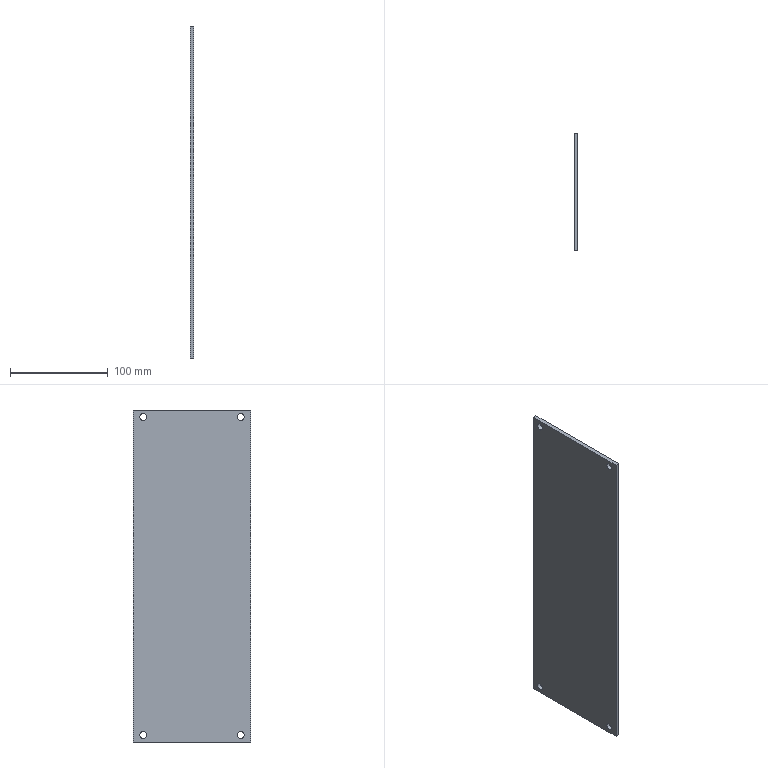Component | NX | HOUSING_COVER | 1 solid | 10 faces | box 4 x 120 x 340 mm | volume 162584 mm3 | plane 6 | cylinder 4 | commonest cylinder face diameters 7 x4
STEP:
#1=CARTESIAN_POINT('',(0.,0.,0.));
#2=DIRECTION('',(0.,0.,1.));
#3=DIRECTION('',(1.,0.,0.));
#4=AXIS2_PLACEMENT_3D('',#1,#2,#3);
#5=CARTESIAN_POINT('',(752.689,-210.302,-955.));
#6=VERTEX_POINT('',#5);
#7=CARTESIAN_POINT('',(752.689,-210.302,-1295.));
#8=VERTEX_POINT('',#7);
#9=CARTESIAN_POINT('',(752.689,-210.302,-955.));
#10=DIRECTION('',(0.,0.,-1.));
#11=VECTOR('',#10,1.);
#12=LINE('',#9,#11);
#13=CARTESIAN_POINT('',(756.689,-210.302,-955.));
#14=DIRECTION('',(0.,1.,0.));
#15=DIRECTION('',(-1.,0.,0.));
#16=AXIS2_PLACEMENT_3D('',#13,#14,#15);
#17=PLANE('',#16);
#18=CARTESIAN_POINT('',(4.,0.));
#19=DIRECTION('',(0.,-1.));
#20=VECTOR('',#19,1.);
#21=LINE('',#18,#20);
#22=(GEOMETRIC_REPRESENTATION_CONTEXT(2)PARAMETRIC_REPRESENTATION_CONTEXT()REPRESENTATION_CONTEXT('',''));
#23=DEFINITIONAL_REPRESENTATION('',(#21),#22);
#24=PCURVE('',#17,#23);
#25=CARTESIAN_POINT('',(752.689,-100.302,-962.));
#26=DIRECTION('',(-1.,0.,0.));
#27=DIRECTION('',(0.,-1.,0.));
#28=AXIS2_PLACEMENT_3D('',#25,#26,#27);
#29=PLANE('',#28);
#30=CARTESIAN_POINT('',(110.,7.));
#31=DIRECTION('',(0.,-1.));
#32=VECTOR('',#31,1.);
#33=LINE('',#30,#32);
#34=(GEOMETRIC_REPRESENTATION_CONTEXT(2)PARAMETRIC_REPRESENTATION_CONTEXT()REPRESENTATION_CONTEXT('',''));
#35=DEFINITIONAL_REPRESENTATION('',(#33),#34);
#36=PCURVE('',#29,#35);
#37=SURFACE_CURVE('',#12,(#24,#36),.PCURVE_S1.);
#38=EDGE_CURVE('',#6,#8,#37,.T.);
#39=ORIENTED_EDGE('',*,*,#38,.T.);
#40=CARTESIAN_POINT('',(756.689,-210.302,-1295.));
#41=VERTEX_POINT('',#40);
#42=CARTESIAN_POINT('',(756.689,-210.302,-1295.));
#43=DIRECTION('',(-1.,0.,0.));
#44=VECTOR('',#43,1.);
#45=LINE('',#42,#44);
#46=CARTESIAN_POINT('',(0.,-340.));
#47=DIRECTION('',(1.,0.));
#48=VECTOR('',#47,1.);
#49=LINE('',#46,#48);
#50=(GEOMETRIC_REPRESENTATION_CONTEXT(2)PARAMETRIC_REPRESENTATION_CONTEXT()REPRESENTATION_CONTEXT('',''));
#51=DEFINITIONAL_REPRESENTATION('',(#49),#50);
#52=PCURVE('',#17,#51);
#53=CARTESIAN_POINT('',(756.689,-210.302,-1295.));
#54=DIRECTION('',(0.,0.,1.));
#55=DIRECTION('',(1.,0.,0.));
#56=AXIS2_PLACEMENT_3D('',#53,#54,#55);
#57=PLANE('',#56);
#58=CARTESIAN_POINT('',(0.,0.));
#59=DIRECTION('',(-1.,0.));
#60=VECTOR('',#59,1.);
#61=LINE('',#58,#60);
#62=(GEOMETRIC_REPRESENTATION_CONTEXT(2)PARAMETRIC_REPRESENTATION_CONTEXT()REPRESENTATION_CONTEXT('',''));
#63=DEFINITIONAL_REPRESENTATION('',(#61),#62);
#64=PCURVE('',#57,#63);
#65=SURFACE_CURVE('',#45,(#52,#64),.PCURVE_S1.);
#66=EDGE_CURVE('',#41,#8,#65,.T.);
#67=ORIENTED_EDGE('',*,*,#66,.F.);
#68=CARTESIAN_POINT('',(756.689,-210.302,-955.));
#69=VERTEX_POINT('',#68);
#70=CARTESIAN_POINT('',(756.689,-210.302,-955.));
#71=DIRECTION('',(0.,0.,-1.));
#72=VECTOR('',#71,1.);
#73=LINE('',#70,#72);
#74=CARTESIAN_POINT('',(0.,0.));
#75=DIRECTION('',(0.,-1.));
#76=VECTOR('',#75,1.);
#77=LINE('',#74,#76);
#78=(GEOMETRIC_REPRESENTATION_CONTEXT(2)PARAMETRIC_REPRESENTATION_CONTEXT()REPRESENTATION_CONTEXT('',''));
#79=DEFINITIONAL_REPRESENTATION('',(#77),#78);
#80=PCURVE('',#17,#79);
#81=CARTESIAN_POINT('',(756.689,-100.302,-962.));
#82=DIRECTION('',(-1.,0.,0.));
#83=DIRECTION('',(0.,-1.,0.));
#84=AXIS2_PLACEMENT_3D('',#81,#82,#83);
#85=PLANE('',#84);
#86=CARTESIAN_POINT('',(110.,7.));
#87=DIRECTION('',(0.,-1.));
#88=VECTOR('',#87,1.);
#89=LINE('',#86,#88);
#90=(GEOMETRIC_REPRESENTATION_CONTEXT(2)PARAMETRIC_REPRESENTATION_CONTEXT()REPRESENTATION_CONTEXT('',''));
#91=DEFINITIONAL_REPRESENTATION('',(#89),#90);
#92=PCURVE('',#85,#91);
#93=SURFACE_CURVE('',#73,(#80,#92),.PCURVE_S1.);
#94=EDGE_CURVE('',#69,#41,#93,.T.);
#95=ORIENTED_EDGE('',*,*,#94,.F.);
#96=CARTESIAN_POINT('',(756.689,-210.302,-955.));
#97=DIRECTION('',(-1.,0.,0.));
#98=VECTOR('',#97,1.);
#99=LINE('',#96,#98);
#100=CARTESIAN_POINT('',(0.,0.));
#101=DIRECTION('',(1.,0.));
#102=VECTOR('',#101,1.);
#103=LINE('',#100,#102);
#104=(GEOMETRIC_REPRESENTATION_CONTEXT(2)PARAMETRIC_REPRESENTATION_CONTEXT()REPRESENTATION_CONTEXT('',''));
#105=DEFINITIONAL_REPRESENTATION('',(#103),#104);
#106=PCURVE('',#17,#105);
#107=CARTESIAN_POINT('',(756.689,-90.302,-955.));
#108=DIRECTION('',(0.,0.,-1.));
#109=DIRECTION('',(-1.,0.,0.));
#110=AXIS2_PLACEMENT_3D('',#107,#108,#109);
#111=PLANE('',#110);
#112=CARTESIAN_POINT('',(0.,-120.));
#113=DIRECTION('',(1.,0.));
#114=VECTOR('',#113,1.);
#115=LINE('',#112,#114);
#116=(GEOMETRIC_REPRESENTATION_CONTEXT(2)PARAMETRIC_REPRESENTATION_CONTEXT()REPRESENTATION_CONTEXT('',''));
#117=DEFINITIONAL_REPRESENTATION('',(#115),#116);
#118=PCURVE('',#111,#117);
#119=SURFACE_CURVE('',#99,(#106,#118),.PCURVE_S1.);
#120=EDGE_CURVE('',#69,#6,#119,.T.);
#121=ORIENTED_EDGE('',*,*,#120,.T.);
#122=EDGE_LOOP('',(#39,#67,#95,#121));
#123=FACE_BOUND('',#122,.T.);
#124=ADVANCED_FACE('',(#123),#17,.F.);
#125=CARTESIAN_POINT('',(752.689,-90.302,-1295.));
#126=VERTEX_POINT('',#125);
#127=CARTESIAN_POINT('',(752.689,-210.302,-1295.));
#128=DIRECTION('',(0.,1.,0.));
#129=VECTOR('',#128,1.);
#130=LINE('',#127,#129);
#131=CARTESIAN_POINT('',(-4.,0.));
#132=DIRECTION('',(0.,1.));
#133=VECTOR('',#132,1.);
#134=LINE('',#131,#133);
#135=(GEOMETRIC_REPRESENTATION_CONTEXT(2)PARAMETRIC_REPRESENTATION_CONTEXT()REPRESENTATION_CONTEXT('',''));
#136=DEFINITIONAL_REPRESENTATION('',(#134),#135);
#137=PCURVE('',#57,#136);
#138=CARTESIAN_POINT('',(110.,-333.));
#139=DIRECTION('',(-1.,0.));
#140=VECTOR('',#139,1.);
#141=LINE('',#138,#140);
#142=(GEOMETRIC_REPRESENTATION_CONTEXT(2)PARAMETRIC_REPRESENTATION_CONTEXT()REPRESENTATION_CONTEXT('',''));
#143=DEFINITIONAL_REPRESENTATION('',(#141),#142);
#144=PCURVE('',#29,#143);
#145=SURFACE_CURVE('',#130,(#137,#144),.PCURVE_S1.);
#146=EDGE_CURVE('',#8,#126,#145,.T.);
#147=ORIENTED_EDGE('',*,*,#146,.T.);
#148=CARTESIAN_POINT('',(756.689,-90.302,-1295.));
#149=VERTEX_POINT('',#148);
#150=CARTESIAN_POINT('',(756.689,-90.302,-1295.));
#151=DIRECTION('',(-1.,0.,0.));
#152=VECTOR('',#151,1.);
#153=LINE('',#150,#152);
#154=CARTESIAN_POINT('',(0.,120.));
#155=DIRECTION('',(-1.,0.));
#156=VECTOR('',#155,1.);
#157=LINE('',#154,#156);
#158=(GEOMETRIC_REPRESENTATION_CONTEXT(2)PARAMETRIC_REPRESENTATION_CONTEXT()REPRESENTATION_CONTEXT('',''));
#159=DEFINITIONAL_REPRESENTATION('',(#157),#158);
#160=PCURVE('',#57,#159);
#161=CARTESIAN_POINT('',(756.689,-90.302,-1295.));
#162=DIRECTION('',(0.,-1.,0.));
#163=DIRECTION('',(1.,0.,0.));
#164=AXIS2_PLACEMENT_3D('',#161,#162,#163);
#165=PLANE('',#164);
#166=CARTESIAN_POINT('',(0.,0.));
#167=DIRECTION('',(-1.,0.));
#168=VECTOR('',#167,1.);
#169=LINE('',#166,#168);
#170=(GEOMETRIC_REPRESENTATION_CONTEXT(2)PARAMETRIC_REPRESENTATION_CONTEXT()REPRESENTATION_CONTEXT('',''));
#171=DEFINITIONAL_REPRESENTATION('',(#169),#170);
#172=PCURVE('',#165,#171);
#173=SURFACE_CURVE('',#153,(#160,#172),.PCURVE_S1.);
#174=EDGE_CURVE('',#149,#126,#173,.T.);
#175=ORIENTED_EDGE('',*,*,#174,.F.);
#176=CARTESIAN_POINT('',(756.689,-210.302,-1295.));
#177=DIRECTION('',(0.,1.,0.));
#178=VECTOR('',#177,1.);
#179=LINE('',#176,#178);
#180=CARTESIAN_POINT('',(0.,0.));
#181=DIRECTION('',(0.,1.));
#182=VECTOR('',#181,1.);
#183=LINE('',#180,#182);
#184=(GEOMETRIC_REPRESENTATION_CONTEXT(2)PARAMETRIC_REPRESENTATION_CONTEXT()REPRESENTATION_CONTEXT('',''));
#185=DEFINITIONAL_REPRESENTATION('',(#183),#184);
#186=PCURVE('',#57,#185);
#187=CARTESIAN_POINT('',(110.,-333.));
#188=DIRECTION('',(-1.,0.));
#189=VECTOR('',#188,1.);
#190=LINE('',#187,#189);
#191=(GEOMETRIC_REPRESENTATION_CONTEXT(2)PARAMETRIC_REPRESENTATION_CONTEXT()REPRESENTATION_CONTEXT('',''));
#192=DEFINITIONAL_REPRESENTATION('',(#190),#191);
#193=PCURVE('',#85,#192);
#194=SURFACE_CURVE('',#179,(#186,#193),.PCURVE_S1.);
#195=EDGE_CURVE('',#41,#149,#194,.T.);
#196=ORIENTED_EDGE('',*,*,#195,.F.);
#197=ORIENTED_EDGE('',*,*,#66,.T.);
#198=EDGE_LOOP('',(#147,#175,#196,#197));
#199=FACE_BOUND('',#198,.T.);
#200=ADVANCED_FACE('',(#199),#57,.F.);
#201=CARTESIAN_POINT('',(752.689,-90.302,-955.));
#202=VERTEX_POINT('',#201);
#203=CARTESIAN_POINT('',(752.689,-90.302,-1295.));
#204=DIRECTION('',(0.,0.,1.));
#205=VECTOR('',#204,1.);
#206=LINE('',#203,#205);
#207=CARTESIAN_POINT('',(-4.,0.));
#208=DIRECTION('',(0.,1.));
#209=VECTOR('',#208,1.);
#210=LINE('',#207,#209);
#211=(GEOMETRIC_REPRESENTATION_CONTEXT(2)PARAMETRIC_REPRESENTATION_CONTEXT()REPRESENTATION_CONTEXT('',''));
#212=DEFINITIONAL_REPRESENTATION('',(#210),#211);
#213=PCURVE('',#165,#212);
#214=CARTESIAN_POINT('',(-10.,-333.));
#215=DIRECTION('',(0.,1.));
#216=VECTOR('',#215,1.);
#217=LINE('',#214,#216);
#218=(GEOMETRIC_REPRESENTATION_CONTEXT(2)PARAMETRIC_REPRESENTATION_CONTEXT()REPRESENTATION_CONTEXT('',''));
#219=DEFINITIONAL_REPRESENTATION('',(#217),#218);
#220=PCURVE('',#29,#219);
#221=SURFACE_CURVE('',#206,(#213,#220),.PCURVE_S1.);
#222=EDGE_CURVE('',#126,#202,#221,.T.);
#223=ORIENTED_EDGE('',*,*,#222,.T.);
#224=CARTESIAN_POINT('',(756.689,-90.302,-955.));
#225=VERTEX_POINT('',#224);
#226=CARTESIAN_POINT('',(756.689,-90.302,-955.));
#227=DIRECTION('',(-1.,0.,0.));
#228=VECTOR('',#227,1.);
#229=LINE('',#226,#228);
#230=CARTESIAN_POINT('',(0.,340.));
#231=DIRECTION('',(-1.,0.));
#232=VECTOR('',#231,1.);
#233=LINE('',#230,#232);
#234=(GEOMETRIC_REPRESENTATION_CONTEXT(2)PARAMETRIC_REPRESENTATION_CONTEXT()REPRESENTATION_CONTEXT('',''));
#235=DEFINITIONAL_REPRESENTATION('',(#233),#234);
#236=PCURVE('',#165,#235);
#237=CARTESIAN_POINT('',(0.,0.));
#238=DIRECTION('',(1.,0.));
#239=VECTOR('',#238,1.);
#240=LINE('',#237,#239);
#241=(GEOMETRIC_REPRESENTATION_CONTEXT(2)PARAMETRIC_REPRESENTATION_CONTEXT()REPRESENTATION_CONTEXT('',''));
#242=DEFINITIONAL_REPRESENTATION('',(#240),#241);
#243=PCURVE('',#111,#242);
#244=SURFACE_CURVE('',#229,(#236,#243),.PCURVE_S1.);
#245=EDGE_CURVE('',#225,#202,#244,.T.);
#246=ORIENTED_EDGE('',*,*,#245,.F.);
#247=CARTESIAN_POINT('',(756.689,-90.302,-1295.));
#248=DIRECTION('',(0.,0.,1.));
#249=VECTOR('',#248,1.);
#250=LINE('',#247,#249);
#251=CARTESIAN_POINT('',(0.,0.));
#252=DIRECTION('',(0.,1.));
#253=VECTOR('',#252,1.);
#254=LINE('',#251,#253);
#255=(GEOMETRIC_REPRESENTATION_CONTEXT(2)PARAMETRIC_REPRESENTATION_CONTEXT()REPRESENTATION_CONTEXT('',''));
#256=DEFINITIONAL_REPRESENTATION('',(#254),#255);
#257=PCURVE('',#165,#256);
#258=CARTESIAN_POINT('',(-10.,-333.));
#259=DIRECTION('',(0.,1.));
#260=VECTOR('',#259,1.);
#261=LINE('',#258,#260);
#262=(GEOMETRIC_REPRESENTATION_CONTEXT(2)PARAMETRIC_REPRESENTATION_CONTEXT()REPRESENTATION_CONTEXT('',''));
#263=DEFINITIONAL_REPRESENTATION('',(#261),#262);
#264=PCURVE('',#85,#263);
#265=SURFACE_CURVE('',#250,(#257,#264),.PCURVE_S1.);
#266=EDGE_CURVE('',#149,#225,#265,.T.);
#267=ORIENTED_EDGE('',*,*,#266,.F.);
#268=ORIENTED_EDGE('',*,*,#174,.T.);
#269=EDGE_LOOP('',(#223,#246,#267,#268));
#270=FACE_BOUND('',#269,.T.);
#271=ADVANCED_FACE('',(#270),#165,.F.);
#272=CARTESIAN_POINT('',(756.689,-196.802,-962.));
#273=VERTEX_POINT('',#272);
#274=CARTESIAN_POINT('',(756.689,-200.302,-962.));
#275=DIRECTION('',(1.,0.,0.));
#276=DIRECTION('',(0.,1.,0.));
#277=AXIS2_PLACEMENT_3D('',#274,#275,#276);
#278=CIRCLE('',#277,3.5);
#279=CARTESIAN_POINT('',(756.689,-200.302,-962.));
#280=DIRECTION('',(-1.,0.,0.));
#281=DIRECTION('',(0.,-1.,0.));
#282=AXIS2_PLACEMENT_3D('',#279,#280,#281);
#283=CYLINDRICAL_SURFACE('',#282,3.5);
#284=CARTESIAN_POINT('',(9.425,0.));
#285=DIRECTION('',(-1.,0.));
#286=VECTOR('',#285,1.);
#287=LINE('',#284,#286);
#288=(GEOMETRIC_REPRESENTATION_CONTEXT(2)PARAMETRIC_REPRESENTATION_CONTEXT()REPRESENTATION_CONTEXT('',''));
#289=DEFINITIONAL_REPRESENTATION('',(#287),#288);
#290=PCURVE('',#283,#289);
#291=CARTESIAN_POINT('',(96.5,0.));
#292=CARTESIAN_POINT('',(96.5,6.062));
#293=CARTESIAN_POINT('',(101.75,3.031));
#294=CARTESIAN_POINT('',(107.,0.));
#295=CARTESIAN_POINT('',(101.75,-3.031));
#296=CARTESIAN_POINT('',(96.5,-6.062));
#297=CARTESIAN_POINT('',(96.5,0.));
#298=(BOUNDED_CURVE()B_SPLINE_CURVE(2,(#291,#292,#293,#294,#295,#296,#297),.UNSPECIFIED.,.T.,.F.)B_SPLINE_CURVE_WITH_KNOTS((1,2,2,2,2,1),(-2.094,0.,2.094,4.189,6.283,8.378),.UNSPECIFIED.)CURVE()GEOMETRIC_REPRESENTATION_ITEM()RATIONAL_B_SPLINE_CURVE((1.,0.5,1.,0.5,1.,0.5,1.))REPRESENTATION_ITEM(''));
#299=(GEOMETRIC_REPRESENTATION_CONTEXT(2)PARAMETRIC_REPRESENTATION_CONTEXT()REPRESENTATION_CONTEXT('',''));
#300=DEFINITIONAL_REPRESENTATION('',(#298),#299);
#301=PCURVE('',#85,#300);
#302=SURFACE_CURVE('',#278,(#290,#301),.PCURVE_S1.);
#303=EDGE_CURVE('',#273,#273,#302,.T.);
#304=ORIENTED_EDGE('',*,*,#303,.F.);
#305=CARTESIAN_POINT('',(752.689,-196.802,-962.));
#306=VERTEX_POINT('',#305);
#307=CARTESIAN_POINT('',(756.689,-196.802,-962.));
#308=CARTESIAN_POINT('',(752.689,-196.802,-962.));
#309=B_SPLINE_CURVE_WITH_KNOTS('',1,(#307,#308),.UNSPECIFIED.,.F.,.F.,(2,2),(0.,4.),.PIECEWISE_BEZIER_KNOTS.);
#310=CARTESIAN_POINT('',(9.425,0.));
#311=DIRECTION('',(0.,1.));
#312=VECTOR('',#311,1.);
#313=LINE('',#310,#312);
#314=(GEOMETRIC_REPRESENTATION_CONTEXT(2)PARAMETRIC_REPRESENTATION_CONTEXT()REPRESENTATION_CONTEXT('',''));
#315=DEFINITIONAL_REPRESENTATION('',(#313),#314);
#316=PCURVE('',#283,#315);
#317=CARTESIAN_POINT('',(3.142,0.));
#318=DIRECTION('',(0.,1.));
#319=VECTOR('',#318,1.);
#320=LINE('',#317,#319);
#321=(GEOMETRIC_REPRESENTATION_CONTEXT(2)PARAMETRIC_REPRESENTATION_CONTEXT()REPRESENTATION_CONTEXT('',''));
#322=DEFINITIONAL_REPRESENTATION('',(#320),#321);
#323=PCURVE('',#283,#322);
#324=SEAM_CURVE('',#309,(#316,#323),.PCURVE_S1.);
#325=EDGE_CURVE('',#273,#306,#324,.T.);
#326=ORIENTED_EDGE('',*,*,#325,.T.);
#327=CARTESIAN_POINT('',(752.689,-200.302,-962.));
#328=DIRECTION('',(1.,0.,0.));
#329=DIRECTION('',(0.,1.,0.));
#330=AXIS2_PLACEMENT_3D('',#327,#328,#329);
#331=CIRCLE('',#330,3.5);
#332=CARTESIAN_POINT('',(9.425,4.));
#333=DIRECTION('',(-1.,0.));
#334=VECTOR('',#333,1.);
#335=LINE('',#332,#334);
#336=(GEOMETRIC_REPRESENTATION_CONTEXT(2)PARAMETRIC_REPRESENTATION_CONTEXT()REPRESENTATION_CONTEXT('',''));
#337=DEFINITIONAL_REPRESENTATION('',(#335),#336);
#338=PCURVE('',#283,#337);
#339=CARTESIAN_POINT('',(96.5,0.));
#340=CARTESIAN_POINT('',(96.5,6.062));
#341=CARTESIAN_POINT('',(101.75,3.031));
#342=CARTESIAN_POINT('',(107.,0.));
#343=CARTESIAN_POINT('',(101.75,-3.031));
#344=CARTESIAN_POINT('',(96.5,-6.062));
#345=CARTESIAN_POINT('',(96.5,0.));
#346=(BOUNDED_CURVE()B_SPLINE_CURVE(2,(#339,#340,#341,#342,#343,#344,#345),.UNSPECIFIED.,.T.,.F.)B_SPLINE_CURVE_WITH_KNOTS((1,2,2,2,2,1),(-2.094,0.,2.094,4.189,6.283,8.378),.UNSPECIFIED.)CURVE()GEOMETRIC_REPRESENTATION_ITEM()RATIONAL_B_SPLINE_CURVE((1.,0.5,1.,0.5,1.,0.5,1.))REPRESENTATION_ITEM(''));
#347=(GEOMETRIC_REPRESENTATION_CONTEXT(2)PARAMETRIC_REPRESENTATION_CONTEXT()REPRESENTATION_CONTEXT('',''));
#348=DEFINITIONAL_REPRESENTATION('',(#346),#347);
#349=PCURVE('',#29,#348);
#350=SURFACE_CURVE('',#331,(#338,#349),.PCURVE_S1.);
#351=EDGE_CURVE('',#306,#306,#350,.T.);
#352=ORIENTED_EDGE('',*,*,#351,.T.);
#353=ORIENTED_EDGE('',*,*,#325,.F.);
#354=EDGE_LOOP('',(#304,#326,#352,#353));
#355=FACE_BOUND('',#354,.F.);
#356=ADVANCED_FACE('',(#355),#283,.F.);
#357=CARTESIAN_POINT('',(756.689,-103.802,-1288.));
#358=VERTEX_POINT('',#357);
#359=CARTESIAN_POINT('',(756.689,-100.302,-1288.));
#360=DIRECTION('',(1.,0.,0.));
#361=DIRECTION('',(0.,-1.,0.));
#362=AXIS2_PLACEMENT_3D('',#359,#360,#361);
#363=CIRCLE('',#362,3.5);
#364=CARTESIAN_POINT('',(756.689,-100.302,-1288.));
#365=DIRECTION('',(-1.,0.,0.));
#366=DIRECTION('',(0.,-1.,0.));
#367=AXIS2_PLACEMENT_3D('',#364,#365,#366);
#368=CYLINDRICAL_SURFACE('',#367,3.5);
#369=CARTESIAN_POINT('',(6.283,0.));
#370=DIRECTION('',(-1.,0.));
#371=VECTOR('',#370,1.);
#372=LINE('',#369,#371);
#373=(GEOMETRIC_REPRESENTATION_CONTEXT(2)PARAMETRIC_REPRESENTATION_CONTEXT()REPRESENTATION_CONTEXT('',''));
#374=DEFINITIONAL_REPRESENTATION('',(#372),#373);
#375=PCURVE('',#368,#374);
#376=CARTESIAN_POINT('',(3.5,-326.));
#377=CARTESIAN_POINT('',(3.5,-332.062));
#378=CARTESIAN_POINT('',(-1.75,-329.031));
#379=CARTESIAN_POINT('',(-7.,-326.));
#380=CARTESIAN_POINT('',(-1.75,-322.969));
#381=CARTESIAN_POINT('',(3.5,-319.938));
#382=CARTESIAN_POINT('',(3.5,-326.));
#383=(BOUNDED_CURVE()B_SPLINE_CURVE(2,(#376,#377,#378,#379,#380,#381,#382),.UNSPECIFIED.,.T.,.F.)B_SPLINE_CURVE_WITH_KNOTS((1,2,2,2,2,1),(-2.094,0.,2.094,4.189,6.283,8.378),.UNSPECIFIED.)CURVE()GEOMETRIC_REPRESENTATION_ITEM()RATIONAL_B_SPLINE_CURVE((1.,0.5,1.,0.5,1.,0.5,1.))REPRESENTATION_ITEM(''));
#384=(GEOMETRIC_REPRESENTATION_CONTEXT(2)PARAMETRIC_REPRESENTATION_CONTEXT()REPRESENTATION_CONTEXT('',''));
#385=DEFINITIONAL_REPRESENTATION('',(#383),#384);
#386=PCURVE('',#85,#385);
#387=SURFACE_CURVE('',#363,(#375,#386),.PCURVE_S1.);
#388=EDGE_CURVE('',#358,#358,#387,.T.);
#389=ORIENTED_EDGE('',*,*,#388,.F.);
#390=CARTESIAN_POINT('',(752.689,-103.802,-1288.));
#391=VERTEX_POINT('',#390);
#392=CARTESIAN_POINT('',(756.689,-103.802,-1288.));
#393=CARTESIAN_POINT('',(752.689,-103.802,-1288.));
#394=B_SPLINE_CURVE_WITH_KNOTS('',1,(#392,#393),.UNSPECIFIED.,.F.,.F.,(2,2),(0.,4.),.PIECEWISE_BEZIER_KNOTS.);
#395=CARTESIAN_POINT('',(6.283,0.));
#396=DIRECTION('',(0.,1.));
#397=VECTOR('',#396,1.);
#398=LINE('',#395,#397);
#399=(GEOMETRIC_REPRESENTATION_CONTEXT(2)PARAMETRIC_REPRESENTATION_CONTEXT()REPRESENTATION_CONTEXT('',''));
#400=DEFINITIONAL_REPRESENTATION('',(#398),#399);
#401=PCURVE('',#368,#400);
#402=CARTESIAN_POINT('',(0.,0.));
#403=DIRECTION('',(0.,1.));
#404=VECTOR('',#403,1.);
#405=LINE('',#402,#404);
#406=(GEOMETRIC_REPRESENTATION_CONTEXT(2)PARAMETRIC_REPRESENTATION_CONTEXT()REPRESENTATION_CONTEXT('',''));
#407=DEFINITIONAL_REPRESENTATION('',(#405),#406);
#408=PCURVE('',#368,#407);
#409=SEAM_CURVE('',#394,(#401,#408),.PCURVE_S1.);
#410=EDGE_CURVE('',#358,#391,#409,.T.);
#411=ORIENTED_EDGE('',*,*,#410,.T.);
#412=CARTESIAN_POINT('',(752.689,-100.302,-1288.));
#413=DIRECTION('',(1.,0.,0.));
#414=DIRECTION('',(0.,-1.,0.));
#415=AXIS2_PLACEMENT_3D('',#412,#413,#414);
#416=CIRCLE('',#415,3.5);
#417=CARTESIAN_POINT('',(6.283,4.));
#418=DIRECTION('',(-1.,0.));
#419=VECTOR('',#418,1.);
#420=LINE('',#417,#419);
#421=(GEOMETRIC_REPRESENTATION_CONTEXT(2)PARAMETRIC_REPRESENTATION_CONTEXT()REPRESENTATION_CONTEXT('',''));
#422=DEFINITIONAL_REPRESENTATION('',(#420),#421);
#423=PCURVE('',#368,#422);
#424=CARTESIAN_POINT('',(3.5,-326.));
#425=CARTESIAN_POINT('',(3.5,-332.062));
#426=CARTESIAN_POINT('',(-1.75,-329.031));
#427=CARTESIAN_POINT('',(-7.,-326.));
#428=CARTESIAN_POINT('',(-1.75,-322.969));
#429=CARTESIAN_POINT('',(3.5,-319.938));
#430=CARTESIAN_POINT('',(3.5,-326.));
#431=(BOUNDED_CURVE()B_SPLINE_CURVE(2,(#424,#425,#426,#427,#428,#429,#430),.UNSPECIFIED.,.T.,.F.)B_SPLINE_CURVE_WITH_KNOTS((1,2,2,2,2,1),(-2.094,0.,2.094,4.189,6.283,8.378),.UNSPECIFIED.)CURVE()GEOMETRIC_REPRESENTATION_ITEM()RATIONAL_B_SPLINE_CURVE((1.,0.5,1.,0.5,1.,0.5,1.))REPRESENTATION_ITEM(''));
#432=(GEOMETRIC_REPRESENTATION_CONTEXT(2)PARAMETRIC_REPRESENTATION_CONTEXT()REPRESENTATION_CONTEXT('',''));
#433=DEFINITIONAL_REPRESENTATION('',(#431),#432);
#434=PCURVE('',#29,#433);
#435=SURFACE_CURVE('',#416,(#423,#434),.PCURVE_S1.);
#436=EDGE_CURVE('',#391,#391,#435,.T.);
#437=ORIENTED_EDGE('',*,*,#436,.T.);
#438=ORIENTED_EDGE('',*,*,#410,.F.);
#439=EDGE_LOOP('',(#389,#411,#437,#438));
#440=FACE_BOUND('',#439,.F.);
#441=ADVANCED_FACE('',(#440),#368,.F.);
#442=CARTESIAN_POINT('',(756.689,-103.802,-962.));
#443=VERTEX_POINT('',#442);
#444=CARTESIAN_POINT('',(756.689,-100.302,-962.));
#445=DIRECTION('',(-1.,0.,0.));
#446=DIRECTION('',(0.,-1.,0.));
#447=AXIS2_PLACEMENT_3D('',#444,#445,#446);
#448=CIRCLE('',#447,3.5);
#449=CARTESIAN_POINT('',(756.689,-100.302,-962.));
#450=DIRECTION('',(-1.,0.,0.));
#451=DIRECTION('',(0.,-1.,0.));
#452=AXIS2_PLACEMENT_3D('',#449,#450,#451);
#453=CYLINDRICAL_SURFACE('',#452,3.5);
#454=CARTESIAN_POINT('',(0.,0.));
#455=DIRECTION('',(1.,0.));
#456=VECTOR('',#455,1.);
#457=LINE('',#454,#456);
#458=(GEOMETRIC_REPRESENTATION_CONTEXT(2)PARAMETRIC_REPRESENTATION_CONTEXT()REPRESENTATION_CONTEXT('',''));
#459=DEFINITIONAL_REPRESENTATION('',(#457),#458);
#460=PCURVE('',#453,#459);
#461=CARTESIAN_POINT('',(0.,0.));
#462=DIRECTION('',(1.,0.));
#463=AXIS2_PLACEMENT_2D('',#461,#462);
#464=CIRCLE('',#463,3.5);
#465=(GEOMETRIC_REPRESENTATION_CONTEXT(2)PARAMETRIC_REPRESENTATION_CONTEXT()REPRESENTATION_CONTEXT('',''));
#466=DEFINITIONAL_REPRESENTATION('',(#464),#465);
#467=PCURVE('',#85,#466);
#468=SURFACE_CURVE('',#448,(#460,#467),.PCURVE_S1.);
#469=EDGE_CURVE('',#443,#443,#468,.T.);
#470=ORIENTED_EDGE('',*,*,#469,.T.);
#471=CARTESIAN_POINT('',(752.689,-103.802,-962.));
#472=VERTEX_POINT('',#471);
#473=CARTESIAN_POINT('',(756.689,-103.802,-962.));
#474=CARTESIAN_POINT('',(752.689,-103.802,-962.));
#475=B_SPLINE_CURVE_WITH_KNOTS('',1,(#473,#474),.UNSPECIFIED.,.F.,.F.,(2,2),(0.,4.),.PIECEWISE_BEZIER_KNOTS.);
#476=CARTESIAN_POINT('',(6.283,0.));
#477=DIRECTION('',(0.,1.));
#478=VECTOR('',#477,1.);
#479=LINE('',#476,#478);
#480=(GEOMETRIC_REPRESENTATION_CONTEXT(2)PARAMETRIC_REPRESENTATION_CONTEXT()REPRESENTATION_CONTEXT('',''));
#481=DEFINITIONAL_REPRESENTATION('',(#479),#480);
#482=PCURVE('',#453,#481);
#483=CARTESIAN_POINT('',(0.,0.));
#484=DIRECTION('',(0.,1.));
#485=VECTOR('',#484,1.);
#486=LINE('',#483,#485);
#487=(GEOMETRIC_REPRESENTATION_CONTEXT(2)PARAMETRIC_REPRESENTATION_CONTEXT()REPRESENTATION_CONTEXT('',''));
#488=DEFINITIONAL_REPRESENTATION('',(#486),#487);
#489=PCURVE('',#453,#488);
#490=SEAM_CURVE('',#475,(#482,#489),.PCURVE_S1.);
#491=EDGE_CURVE('',#443,#472,#490,.T.);
#492=ORIENTED_EDGE('',*,*,#491,.T.);
#493=CARTESIAN_POINT('',(752.689,-100.302,-962.));
#494=DIRECTION('',(-1.,0.,0.));
#495=DIRECTION('',(0.,-1.,0.));
#496=AXIS2_PLACEMENT_3D('',#493,#494,#495);
#497=CIRCLE('',#496,3.5);
#498=CARTESIAN_POINT('',(0.,4.));
#499=DIRECTION('',(1.,0.));
#500=VECTOR('',#499,1.);
#501=LINE('',#498,#500);
#502=(GEOMETRIC_REPRESENTATION_CONTEXT(2)PARAMETRIC_REPRESENTATION_CONTEXT()REPRESENTATION_CONTEXT('',''));
#503=DEFINITIONAL_REPRESENTATION('',(#501),#502);
#504=PCURVE('',#453,#503);
#505=CARTESIAN_POINT('',(0.,0.));
#506=DIRECTION('',(1.,0.));
#507=AXIS2_PLACEMENT_2D('',#505,#506);
#508=CIRCLE('',#507,3.5);
#509=(GEOMETRIC_REPRESENTATION_CONTEXT(2)PARAMETRIC_REPRESENTATION_CONTEXT()REPRESENTATION_CONTEXT('',''));
#510=DEFINITIONAL_REPRESENTATION('',(#508),#509);
#511=PCURVE('',#29,#510);
#512=SURFACE_CURVE('',#497,(#504,#511),.PCURVE_S1.);
#513=EDGE_CURVE('',#472,#472,#512,.T.);
#514=ORIENTED_EDGE('',*,*,#513,.F.);
#515=ORIENTED_EDGE('',*,*,#491,.F.);
#516=EDGE_LOOP('',(#470,#492,#514,#515));
#517=FACE_BOUND('',#516,.F.);
#518=ADVANCED_FACE('',(#517),#453,.F.);
#519=CARTESIAN_POINT('',(752.689,-90.302,-955.));
#520=DIRECTION('',(0.,-1.,0.));
#521=VECTOR('',#520,1.);
#522=LINE('',#519,#521);
#523=CARTESIAN_POINT('',(4.,0.));
#524=DIRECTION('',(0.,-1.));
#525=VECTOR('',#524,1.);
#526=LINE('',#523,#525);
#527=(GEOMETRIC_REPRESENTATION_CONTEXT(2)PARAMETRIC_REPRESENTATION_CONTEXT()REPRESENTATION_CONTEXT('',''));
#528=DEFINITIONAL_REPRESENTATION('',(#526),#527);
#529=PCURVE('',#111,#528);
#530=CARTESIAN_POINT('',(-10.,7.));
#531=DIRECTION('',(1.,0.));
#532=VECTOR('',#531,1.);
#533=LINE('',#530,#532);
#534=(GEOMETRIC_REPRESENTATION_CONTEXT(2)PARAMETRIC_REPRESENTATION_CONTEXT()REPRESENTATION_CONTEXT('',''));
#535=DEFINITIONAL_REPRESENTATION('',(#533),#534);
#536=PCURVE('',#29,#535);
#537=SURFACE_CURVE('',#522,(#529,#536),.PCURVE_S1.);
#538=EDGE_CURVE('',#202,#6,#537,.T.);
#539=ORIENTED_EDGE('',*,*,#538,.T.);
#540=ORIENTED_EDGE('',*,*,#120,.F.);
#541=CARTESIAN_POINT('',(756.689,-90.302,-955.));
#542=DIRECTION('',(0.,-1.,0.));
#543=VECTOR('',#542,1.);
#544=LINE('',#541,#543);
#545=CARTESIAN_POINT('',(0.,0.));
#546=DIRECTION('',(0.,-1.));
#547=VECTOR('',#546,1.);
#548=LINE('',#545,#547);
#549=(GEOMETRIC_REPRESENTATION_CONTEXT(2)PARAMETRIC_REPRESENTATION_CONTEXT()REPRESENTATION_CONTEXT('',''));
#550=DEFINITIONAL_REPRESENTATION('',(#548),#549);
#551=PCURVE('',#111,#550);
#552=CARTESIAN_POINT('',(-10.,7.));
#553=DIRECTION('',(1.,0.));
#554=VECTOR('',#553,1.);
#555=LINE('',#552,#554);
#556=(GEOMETRIC_REPRESENTATION_CONTEXT(2)PARAMETRIC_REPRESENTATION_CONTEXT()REPRESENTATION_CONTEXT('',''));
#557=DEFINITIONAL_REPRESENTATION('',(#555),#556);
#558=PCURVE('',#85,#557);
#559=SURFACE_CURVE('',#544,(#551,#558),.PCURVE_S1.);
#560=EDGE_CURVE('',#225,#69,#559,.T.);
#561=ORIENTED_EDGE('',*,*,#560,.F.);
#562=ORIENTED_EDGE('',*,*,#245,.T.);
#563=EDGE_LOOP('',(#539,#540,#561,#562));
#564=FACE_BOUND('',#563,.T.);
#565=ADVANCED_FACE('',(#564),#111,.F.);
#566=CARTESIAN_POINT('',(756.689,-196.802,-1288.));
#567=VERTEX_POINT('',#566);
#568=CARTESIAN_POINT('',(756.689,-200.302,-1288.));
#569=DIRECTION('',(-1.,0.,0.));
#570=DIRECTION('',(0.,1.,0.));
#571=AXIS2_PLACEMENT_3D('',#568,#569,#570);
#572=CIRCLE('',#571,3.5);
#573=CARTESIAN_POINT('',(756.689,-200.302,-1288.));
#574=DIRECTION('',(-1.,0.,0.));
#575=DIRECTION('',(0.,-1.,0.));
#576=AXIS2_PLACEMENT_3D('',#573,#574,#575);
#577=CYLINDRICAL_SURFACE('',#576,3.5);
#578=CARTESIAN_POINT('',(3.142,0.));
#579=DIRECTION('',(1.,0.));
#580=VECTOR('',#579,1.);
#581=LINE('',#578,#580);
#582=(GEOMETRIC_REPRESENTATION_CONTEXT(2)PARAMETRIC_REPRESENTATION_CONTEXT()REPRESENTATION_CONTEXT('',''));
#583=DEFINITIONAL_REPRESENTATION('',(#581),#582);
#584=PCURVE('',#577,#583);
#585=CARTESIAN_POINT('',(100.,-326.));
#586=DIRECTION('',(-1.,0.));
#587=AXIS2_PLACEMENT_2D('',#585,#586);
#588=CIRCLE('',#587,3.5);
#589=(GEOMETRIC_REPRESENTATION_CONTEXT(2)PARAMETRIC_REPRESENTATION_CONTEXT()REPRESENTATION_CONTEXT('',''));
#590=DEFINITIONAL_REPRESENTATION('',(#588),#589);
#591=PCURVE('',#85,#590);
#592=SURFACE_CURVE('',#572,(#584,#591),.PCURVE_S1.);
#593=EDGE_CURVE('',#567,#567,#592,.T.);
#594=ORIENTED_EDGE('',*,*,#593,.T.);
#595=CARTESIAN_POINT('',(752.689,-196.802,-1288.));
#596=VERTEX_POINT('',#595);
#597=CARTESIAN_POINT('',(756.689,-196.802,-1288.));
#598=CARTESIAN_POINT('',(752.689,-196.802,-1288.));
#599=B_SPLINE_CURVE_WITH_KNOTS('',1,(#597,#598),.UNSPECIFIED.,.F.,.F.,(2,2),(0.,4.),.PIECEWISE_BEZIER_KNOTS.);
#600=CARTESIAN_POINT('',(9.425,0.));
#601=DIRECTION('',(0.,1.));
#602=VECTOR('',#601,1.);
#603=LINE('',#600,#602);
#604=(GEOMETRIC_REPRESENTATION_CONTEXT(2)PARAMETRIC_REPRESENTATION_CONTEXT()REPRESENTATION_CONTEXT('',''));
#605=DEFINITIONAL_REPRESENTATION('',(#603),#604);
#606=PCURVE('',#577,#605);
#607=CARTESIAN_POINT('',(3.142,0.));
#608=DIRECTION('',(0.,1.));
#609=VECTOR('',#608,1.);
#610=LINE('',#607,#609);
#611=(GEOMETRIC_REPRESENTATION_CONTEXT(2)PARAMETRIC_REPRESENTATION_CONTEXT()REPRESENTATION_CONTEXT('',''));
#612=DEFINITIONAL_REPRESENTATION('',(#610),#611);
#613=PCURVE('',#577,#612);
#614=SEAM_CURVE('',#599,(#606,#613),.PCURVE_S1.);
#615=EDGE_CURVE('',#567,#596,#614,.T.);
#616=ORIENTED_EDGE('',*,*,#615,.T.);
#617=CARTESIAN_POINT('',(752.689,-200.302,-1288.));
#618=DIRECTION('',(-1.,0.,0.));
#619=DIRECTION('',(0.,1.,0.));
#620=AXIS2_PLACEMENT_3D('',#617,#618,#619);
#621=CIRCLE('',#620,3.5);
#622=CARTESIAN_POINT('',(3.142,4.));
#623=DIRECTION('',(1.,0.));
#624=VECTOR('',#623,1.);
#625=LINE('',#622,#624);
#626=(GEOMETRIC_REPRESENTATION_CONTEXT(2)PARAMETRIC_REPRESENTATION_CONTEXT()REPRESENTATION_CONTEXT('',''));
#627=DEFINITIONAL_REPRESENTATION('',(#625),#626);
#628=PCURVE('',#577,#627);
#629=CARTESIAN_POINT('',(100.,-326.));
#630=DIRECTION('',(-1.,0.));
#631=AXIS2_PLACEMENT_2D('',#629,#630);
#632=CIRCLE('',#631,3.5);
#633=(GEOMETRIC_REPRESENTATION_CONTEXT(2)PARAMETRIC_REPRESENTATION_CONTEXT()REPRESENTATION_CONTEXT('',''));
#634=DEFINITIONAL_REPRESENTATION('',(#632),#633);
#635=PCURVE('',#29,#634);
#636=SURFACE_CURVE('',#621,(#628,#635),.PCURVE_S1.);
#637=EDGE_CURVE('',#596,#596,#636,.T.);
#638=ORIENTED_EDGE('',*,*,#637,.F.);
#639=ORIENTED_EDGE('',*,*,#615,.F.);
#640=EDGE_LOOP('',(#594,#616,#638,#639));
#641=FACE_BOUND('',#640,.F.);
#642=ADVANCED_FACE('',(#641),#577,.F.);
#643=ORIENTED_EDGE('',*,*,#94,.T.);
#644=ORIENTED_EDGE('',*,*,#195,.T.);
#645=ORIENTED_EDGE('',*,*,#266,.T.);
#646=ORIENTED_EDGE('',*,*,#560,.T.);
#647=EDGE_LOOP('',(#643,#644,#645,#646));
#648=FACE_BOUND('',#647,.T.);
#649=ORIENTED_EDGE('',*,*,#469,.T.);
#650=EDGE_LOOP('',(#649));
#651=FACE_BOUND('',#650,.T.);
#652=ORIENTED_EDGE('',*,*,#388,.F.);
#653=EDGE_LOOP('',(#652));
#654=FACE_BOUND('',#653,.T.);
#655=ORIENTED_EDGE('',*,*,#303,.F.);
#656=EDGE_LOOP('',(#655));
#657=FACE_BOUND('',#656,.T.);
#658=ORIENTED_EDGE('',*,*,#593,.T.);
#659=EDGE_LOOP('',(#658));
#660=FACE_BOUND('',#659,.T.);
#661=ADVANCED_FACE('',(#648,#651,#654,#657,#660),#85,.F.);
#662=ORIENTED_EDGE('',*,*,#38,.F.);
#663=ORIENTED_EDGE('',*,*,#538,.F.);
#664=ORIENTED_EDGE('',*,*,#222,.F.);
#665=ORIENTED_EDGE('',*,*,#146,.F.);
#666=EDGE_LOOP('',(#662,#663,#664,#665));
#667=FACE_BOUND('',#666,.T.);
#668=ORIENTED_EDGE('',*,*,#513,.F.);
#669=EDGE_LOOP('',(#668));
#670=FACE_BOUND('',#669,.T.);
#671=ORIENTED_EDGE('',*,*,#436,.T.);
#672=EDGE_LOOP('',(#671));
#673=FACE_BOUND('',#672,.T.);
#674=ORIENTED_EDGE('',*,*,#351,.T.);
#675=EDGE_LOOP('',(#674));
#676=FACE_BOUND('',#675,.T.);
#677=ORIENTED_EDGE('',*,*,#637,.F.);
#678=EDGE_LOOP('',(#677));
#679=FACE_BOUND('',#678,.T.);
#680=ADVANCED_FACE('',(#667,#670,#673,#676,#679),#29,.T.);
#681=CLOSED_SHELL('',(#124,#200,#271,#356,#441,#518,#565,#642,#661,#680));
#682=MANIFOLD_SOLID_BREP('',#681);
#683=(LENGTH_UNIT()NAMED_UNIT(*)SI_UNIT(.MILLI.,.METRE.));
#684=UNCERTAINTY_MEASURE_WITH_UNIT(LENGTH_MEASURE(0.000005),#683,'','');
#685=(NAMED_UNIT(*)PLANE_ANGLE_UNIT()SI_UNIT($,.RADIAN.));
#686=(NAMED_UNIT(*)SI_UNIT($,.STERADIAN.)SOLID_ANGLE_UNIT());
#687=(GEOMETRIC_REPRESENTATION_CONTEXT(3)GLOBAL_UNCERTAINTY_ASSIGNED_CONTEXT((#684))GLOBAL_UNIT_ASSIGNED_CONTEXT((#683,#685,#686))REPRESENTATION_CONTEXT('',''));
#688=ADVANCED_BREP_SHAPE_REPRESENTATION('',(#4,#682),#687);